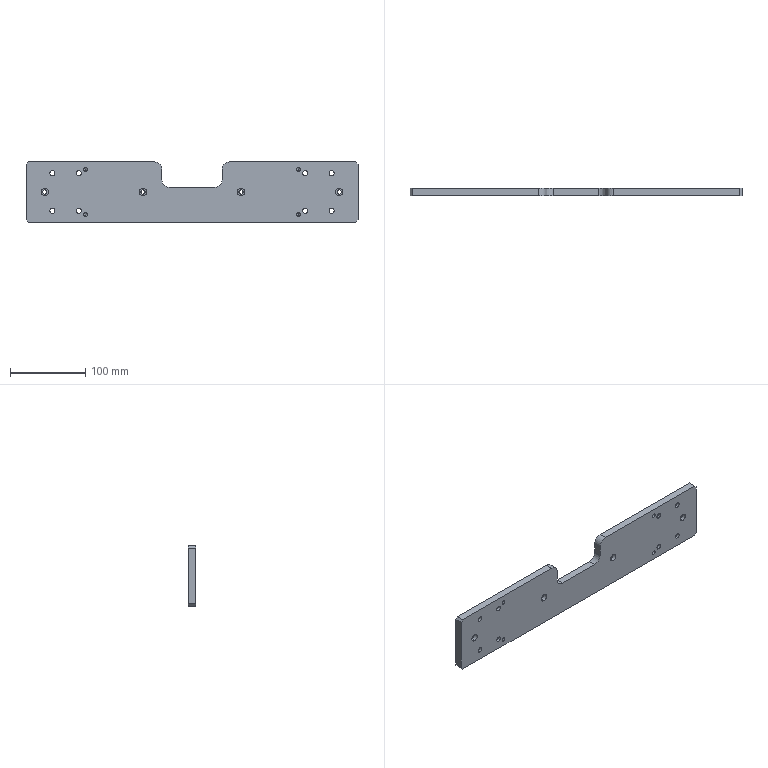Component | SolidWorks | 002MaterialPickingModuleA-1_J-020-1 | 1 solid | 94 faces | box 440 x 10 x 80 mm | volume 315968 mm3 | cylinder 60 | plane 26 | cone 8 | commonest cylinder face diameters 11 x16 6.6 x16 5 x8 10 x8 5.5 x8 20 x4 | material 45
build123d program:
from build123d import *

# Parameters (mm, degrees)
SKETCH1_W                                       = 440
SKETCH1_H                                       = 80
BOSS_EXTRUDE1_DEPTH                             = 10
CHAMFER1_SIZE                                   = 3
M6_HEX_SOCKET_HEAD_CAP_SCREW_CBORE1_D           = 6.6
M6_HEX_SOCKET_HEAD_CAP_SCREW_CBORE1_CBORE_D     = 11
M6_HEX_SOCKET_HEAD_CAP_SCREW_CBORE1_CBORE_DEPTH = 6.4
SKETCH4_W                                       = 80
SKETCH4_H                                       = 68
CUT_EXTRUDE1_DEPTH                              = 224.83
FILLET1_R                                       = 10
M5_HEX_SOCKET_HEAD_CAP_SCREW_CBORE1_D           = 5.5
M5_HEX_SOCKET_HEAD_CAP_SCREW_CBORE1_CBORE_D     = 10
M5_HEX_SOCKET_HEAD_CAP_SCREW_CBORE1_CBORE_DEPTH = 5.4
SIZE_MM_DOWEL_PIN_HOLE1_D                       = 5
SIZE_MM_DOWEL_PIN_HOLE1_DEPTH                   = 8
SIZE_MM_DOWEL_PIN_HOLE1_TIP                     = 1.502


with BuildPart() as part:
    # Sketch1 → Boss-Extrude1 (new body)
    with BuildSketch(Plane(origin=(0, 0, 0), x_dir=(1, 0, 0), z_dir=(0, 1, 0))):
        Rectangle(SKETCH1_W, SKETCH1_H)
    extrude(amount=BOSS_EXTRUDE1_DEPTH)

    # Chamfer1
    chamfer1_edges = [part.edges().sort_by_distance(p)[0] for p in [
        (-220, 5, -40),
        (220, 5, -40),
        (220, 5, 40),
        (-220, 5, 40),
    ]]
    chamfer(chamfer1_edges, length=CHAMFER1_SIZE)

    # M6 Hex Socket Head Cap Screw CBORE1 (through all)
    with Locations(Plane(origin=(0, 10, 0), x_dir=(1, 0, 0), z_dir=(0, 1, 0))):
        with Locations((-185, 25), (-185, -25), (-150, 25), (-150, -25), (150, 25), (150, -25), (185, 25), (185, -25)):
            CounterBoreHole(M6_HEX_SOCKET_HEAD_CAP_SCREW_CBORE1_D / 2, M6_HEX_SOCKET_HEAD_CAP_SCREW_CBORE1_CBORE_D / 2, M6_HEX_SOCKET_HEAD_CAP_SCREW_CBORE1_CBORE_DEPTH)

    # Sketch4 → Cut-Extrude1 (cut, through all)
    with BuildSketch(Plane(origin=(0, 10, 0), x_dir=(1, 0, 0), z_dir=(0, 1, 0))):
        with Locations((0, -40)):
            Rectangle(SKETCH4_W, SKETCH4_H)
    extrude(amount=-CUT_EXTRUDE1_DEPTH, mode=Mode.SUBTRACT)

    # Fillet1
    fillet1_edges = [part.edges().sort_by_distance(p)[0] for p in [
        (-40, 5, 40),
        (40, 5, 40),
        (40, 5, 6),
        (-40, 5, 6),
    ]]
    fillet(fillet1_edges, radius=FILLET1_R)

    # M5 Hex Socket Head Cap Screw CBORE1 (through all)
    with Locations(Plane(origin=(0, 0, 0), x_dir=(-1, 0, 0), z_dir=(0, -1, 0))):
        with Locations((-195, 0), (-65, 0), (65, 0), (195, 0)):
            CounterBoreHole(M5_HEX_SOCKET_HEAD_CAP_SCREW_CBORE1_D / 2, M5_HEX_SOCKET_HEAD_CAP_SCREW_CBORE1_CBORE_D / 2, M5_HEX_SOCKET_HEAD_CAP_SCREW_CBORE1_CBORE_DEPTH)

    # Size mm Dowel Pin Hole1
    with Locations(Plane(origin=(0, 0, 0), x_dir=(-1, 0, 0), z_dir=(0, -1, 0))):
        with Locations((141, -30), (141, 30), (-141, -30), (-141, 30)):
            Hole(SIZE_MM_DOWEL_PIN_HOLE1_D / 2, depth=SIZE_MM_DOWEL_PIN_HOLE1_DEPTH)
            with Locations((0, 0, -(SIZE_MM_DOWEL_PIN_HOLE1_DEPTH + SIZE_MM_DOWEL_PIN_HOLE1_TIP / 2))):  # 118° drill point
                Cone(0, SIZE_MM_DOWEL_PIN_HOLE1_D / 2, SIZE_MM_DOWEL_PIN_HOLE1_TIP, mode=Mode.SUBTRACT)


solid = part.part

# Placed as in the assembly
solid = solid.moved(Location((220.325, 61.019, 422.231), (0, 0, 0)))